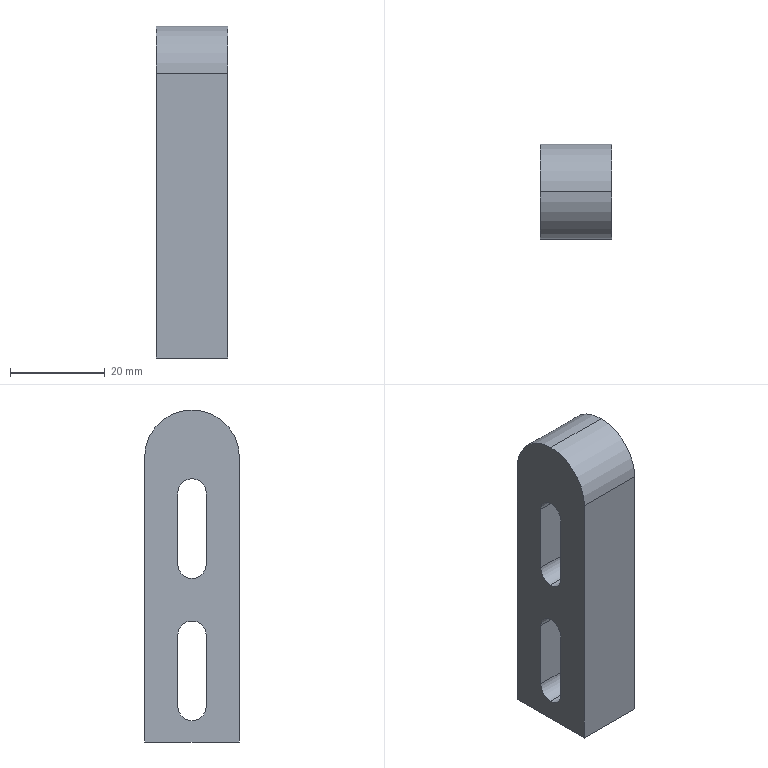Component | SolidWorks | GuideMechanism-1_LimitPlate1-1 | 1 solid | 29 faces | box 15 x 20 x 70 mm | volume 16005 mm3 | plane 15 | cylinder 14 | commonest cylinder face diameters 9 x6 6 x6 20 x2
build123d program:
from build123d import *

# Parameters (mm, degrees)
SKETCH1_W           = 70
SKETCH1_H           = 20
BOSS_EXTRUDE1_DEPTH = 15
FILLET1_RADIUS      = 10
FILLET1_LENGTH      = 15
CUT_EXTRUDE1_DEPTH  = 40.37
CUT_EXTRUDE2_DEPTH  = 5


with BuildPart() as part:
    # Sketch1 → Boss-Extrude1 (new body)
    with BuildSketch(Plane.XY):
        Rectangle(SKETCH1_W, SKETCH1_H)
    extrude(amount=BOSS_EXTRUDE1_DEPTH)

    # Fillet1: full round fillet: the end face becomes a half cylinder, R = half its width
    fillet1_face = Plane((-35, 0, 7.5), x_dir=(0, 0, 1), z_dir=(-1, 0, 0))  # on the end face: x along it, z out of the body
    fillet1_slab = fillet1_face.offset(-FILLET1_RADIUS / 2) * Box(FILLET1_LENGTH, 2 * FILLET1_RADIUS, FILLET1_RADIUS, mode=Mode.PRIVATE)  # the body's end, R deep
    fillet1_round = Plane((-25, 0, 7.5), x_dir=(-1, 0, 0), z_dir=(0, 0, 1)) * Cylinder(FILLET1_RADIUS, FILLET1_LENGTH, mode=Mode.PRIVATE)  # its axis R under the face
    add(fillet1_slab - fillet1_round, mode=Mode.SUBTRACT)

    # Sketch4 → Cut-Extrude1 (cut, through all)
    with BuildSketch(Plane.XY.offset(15)):
        with BuildLine():
            Line((-17.5, 3), (-2.5, 3))
            ThreePointArc((-2.5, 3), (0.5, 0), (-2.5, -3))
            Line((-2.5, -3), (-17.5, -3))
            ThreePointArc((-17.5, -3), (-20.5, 0), (-17.5, 3))
        make_face()
        with BuildLine():
            Line((12.5, 3), (27.5, 3))
            ThreePointArc((27.5, 3), (30.5, 0), (27.5, -3))
            Line((27.5, -3), (12.5, -3))
            ThreePointArc((12.5, -3), (9.5, 0), (12.5, 3))
        make_face()
    extrude(amount=-CUT_EXTRUDE1_DEPTH, mode=Mode.SUBTRACT)

    # Sketch5 → Cut-Extrude2 (cut)
    with BuildSketch(Plane.XY.offset(15)):
        with BuildLine():
            Line((-17.5, 4.5), (-2.5, 4.5))
            ThreePointArc((-2.5, 4.5), (2, 0), (-2.5, -4.5))
            Line((-2.5, -4.5), (-17.5, -4.5))
            ThreePointArc((-17.5, -4.5), (-22, 0), (-17.5, 4.5))
        make_face()
        with BuildLine():
            Line((12.5, 4.5), (27.5, 4.5))
            ThreePointArc((27.5, 4.5), (32, 0), (27.5, -4.5))
            Line((27.5, -4.5), (12.5, -4.5))
            ThreePointArc((12.5, -4.5), (8, 0), (12.5, 4.5))
        make_face()
    extrude(amount=-CUT_EXTRUDE2_DEPTH, mode=Mode.SUBTRACT)


solid = part.part

# Placed as in the assembly
solid = solid.moved(Location((-513.272, -588.766, 1357), (0, 90, 0)))
STEP:
#1=COLOUR_RGB('',0.7922,0.8196,0.9333);
#2=FILL_AREA_STYLE_COLOUR('',#1);
#3=FILL_AREA_STYLE('',(#2));
#4=SURFACE_STYLE_FILL_AREA(#3);
#5=SURFACE_SIDE_STYLE('',(#4));
#6=SURFACE_STYLE_USAGE(.BOTH.,#5);
#7=PRESENTATION_STYLE_ASSIGNMENT((#6));
#8=CARTESIAN_POINT('',(-19.814,-23.18,52.165));
#9=VERTEX_POINT('',#8);
#10=CARTESIAN_POINT('',(-19.814,-23.003,52.343));
#11=VERTEX_POINT('',#10);
#12=CARTESIAN_POINT('',(-19.814,-23.18,52.343));
#13=DIRECTION('',(1.,0.,0.));
#14=DIRECTION('',(0.,0.,-1.));
#15=AXIS2_PLACEMENT_3D('',#12,#13,#14);
#16=CIRCLE('',#15,0.1772);
#17=EDGE_CURVE('',#9,#11,#16,.T.);
#18=ORIENTED_EDGE('',*,*,#17,.F.);
#19=CARTESIAN_POINT('',(-19.617,-23.18,52.165));
#20=VERTEX_POINT('',#19);
#21=CARTESIAN_POINT('',(-19.814,-23.18,52.165));
#22=DIRECTION('',(1.,0.,0.));
#23=VECTOR('',#22,39.37);
#24=LINE('',#21,#23);
#25=EDGE_CURVE('',#9,#20,#24,.T.);
#26=ORIENTED_EDGE('',*,*,#25,.T.);
#27=CARTESIAN_POINT('',(-19.617,-23.003,52.343));
#28=VERTEX_POINT('',#27);
#29=CARTESIAN_POINT('',(-19.617,-23.18,52.343));
#30=DIRECTION('',(1.,0.,0.));
#31=DIRECTION('',(0.,0.,-1.));
#32=AXIS2_PLACEMENT_3D('',#29,#30,#31);
#33=CIRCLE('',#32,0.1772);
#34=EDGE_CURVE('',#20,#28,#33,.T.);
#35=ORIENTED_EDGE('',*,*,#34,.T.);
#36=CARTESIAN_POINT('',(-19.814,-23.003,52.343));
#37=DIRECTION('',(1.,0.,0.));
#38=VECTOR('',#37,39.37);
#39=LINE('',#36,#38);
#40=EDGE_CURVE('',#11,#28,#39,.T.);
#41=ORIENTED_EDGE('',*,*,#40,.F.);
#42=EDGE_LOOP('',(#18,#26,#35,#41));
#43=FACE_OUTER_BOUND('',#42,.T.);
#44=CARTESIAN_POINT('',(-19.814,-23.18,52.343));
#45=DIRECTION('',(1.,0.,0.));
#46=DIRECTION('',(0.,0.,-1.));
#47=AXIS2_PLACEMENT_3D('',#44,#45,#46);
#48=CYLINDRICAL_SURFACE('',#47,0.1772);
#49=ADVANCED_FACE('',(#43),#48,.F.);
#50=CARTESIAN_POINT('',(-19.814,-23.18,53.346));
#51=VERTEX_POINT('',#50);
#52=CARTESIAN_POINT('',(-19.814,-23.003,53.524));
#53=VERTEX_POINT('',#52);
#54=CARTESIAN_POINT('',(-19.814,-23.18,53.524));
#55=DIRECTION('',(1.,0.,0.));
#56=DIRECTION('',(0.,0.,-1.));
#57=AXIS2_PLACEMENT_3D('',#54,#55,#56);
#58=CIRCLE('',#57,0.1772);
#59=EDGE_CURVE('',#51,#53,#58,.T.);
#60=ORIENTED_EDGE('',*,*,#59,.F.);
#61=CARTESIAN_POINT('',(-19.617,-23.18,53.346));
#62=VERTEX_POINT('',#61);
#63=CARTESIAN_POINT('',(-19.814,-23.18,53.346));
#64=DIRECTION('',(1.,0.,0.));
#65=VECTOR('',#64,39.37);
#66=LINE('',#63,#65);
#67=EDGE_CURVE('',#51,#62,#66,.T.);
#68=ORIENTED_EDGE('',*,*,#67,.T.);
#69=CARTESIAN_POINT('',(-19.617,-23.003,53.524));
#70=VERTEX_POINT('',#69);
#71=CARTESIAN_POINT('',(-19.617,-23.18,53.524));
#72=DIRECTION('',(1.,0.,0.));
#73=DIRECTION('',(0.,0.,-1.));
#74=AXIS2_PLACEMENT_3D('',#71,#72,#73);
#75=CIRCLE('',#74,0.1772);
#76=EDGE_CURVE('',#62,#70,#75,.T.);
#77=ORIENTED_EDGE('',*,*,#76,.T.);
#78=CARTESIAN_POINT('',(-19.814,-23.003,53.524));
#79=DIRECTION('',(1.,0.,0.));
#80=VECTOR('',#79,39.37);
#81=LINE('',#78,#80);
#82=EDGE_CURVE('',#53,#70,#81,.T.);
#83=ORIENTED_EDGE('',*,*,#82,.F.);
#84=EDGE_LOOP('',(#60,#68,#77,#83));
#85=FACE_OUTER_BOUND('',#84,.T.);
#86=CARTESIAN_POINT('',(-19.814,-23.18,53.524));
#87=DIRECTION('',(1.,0.,0.));
#88=DIRECTION('',(0.,0.,-1.));
#89=AXIS2_PLACEMENT_3D('',#86,#87,#88);
#90=CYLINDRICAL_SURFACE('',#89,0.1772);
#91=ADVANCED_FACE('',(#85),#90,.F.);
#92=CARTESIAN_POINT('',(-19.617,-23.18,54.803));
#93=VERTEX_POINT('',#92);
#94=CARTESIAN_POINT('',(-19.617,-23.573,54.409));
#95=VERTEX_POINT('',#94);
#96=CARTESIAN_POINT('',(-19.617,-23.18,54.409));
#97=DIRECTION('',(1.,0.,0.));
#98=DIRECTION('',(0.,0.,1.));
#99=AXIS2_PLACEMENT_3D('',#96,#97,#98);
#100=CIRCLE('',#99,0.3937);
#101=EDGE_CURVE('',#93,#95,#100,.T.);
#102=ORIENTED_EDGE('',*,*,#101,.F.);
#103=CARTESIAN_POINT('',(-20.208,-23.18,54.803));
#104=VERTEX_POINT('',#103);
#105=CARTESIAN_POINT('',(-20.208,-23.18,54.803));
#106=DIRECTION('',(-1.,0.,0.));
#107=VECTOR('',#106,39.37);
#108=LINE('',#105,#107);
#109=EDGE_CURVE('',#93,#104,#108,.T.);
#110=ORIENTED_EDGE('',*,*,#109,.T.);
#111=CARTESIAN_POINT('',(-20.208,-23.573,54.409));
#112=VERTEX_POINT('',#111);
#113=CARTESIAN_POINT('',(-20.208,-23.18,54.409));
#114=DIRECTION('',(-1.,0.,0.));
#115=DIRECTION('',(0.,0.,1.));
#116=AXIS2_PLACEMENT_3D('',#113,#114,#115);
#117=CIRCLE('',#116,0.3937);
#118=EDGE_CURVE('',#112,#104,#117,.T.);
#119=ORIENTED_EDGE('',*,*,#118,.F.);
#120=CARTESIAN_POINT('',(-19.617,-23.573,54.409));
#121=DIRECTION('',(-1.,0.,0.));
#122=VECTOR('',#121,39.37);
#123=LINE('',#120,#122);
#124=EDGE_CURVE('',#95,#112,#123,.T.);
#125=ORIENTED_EDGE('',*,*,#124,.F.);
#126=EDGE_LOOP('',(#102,#110,#119,#125));
#127=FACE_OUTER_BOUND('',#126,.T.);
#128=CARTESIAN_POINT('',(-20.208,-23.18,54.409));
#129=DIRECTION('',(-1.,0.,0.));
#130=DIRECTION('',(0.,0.,1.));
#131=AXIS2_PLACEMENT_3D('',#128,#129,#130);
#132=CYLINDRICAL_SURFACE('',#131,0.3937);
#133=ADVANCED_FACE('',(#127),#132,.T.);
#134=CARTESIAN_POINT('',(-20.208,-23.18,53.406));
#135=VERTEX_POINT('',#134);
#136=CARTESIAN_POINT('',(-20.208,-23.062,53.524));
#137=VERTEX_POINT('',#136);
#138=CARTESIAN_POINT('',(-20.208,-23.18,53.524));
#139=DIRECTION('',(1.,0.,0.));
#140=DIRECTION('',(0.,0.,-1.));
#141=AXIS2_PLACEMENT_3D('',#138,#139,#140);
#142=CIRCLE('',#141,0.1181);
#143=EDGE_CURVE('',#135,#137,#142,.T.);
#144=ORIENTED_EDGE('',*,*,#143,.F.);
#145=CARTESIAN_POINT('',(-19.814,-23.18,53.406));
#146=VERTEX_POINT('',#145);
#147=CARTESIAN_POINT('',(-20.208,-23.18,53.406));
#148=DIRECTION('',(1.,0.,0.));
#149=VECTOR('',#148,39.37);
#150=LINE('',#147,#149);
#151=EDGE_CURVE('',#135,#146,#150,.T.);
#152=ORIENTED_EDGE('',*,*,#151,.T.);
#153=CARTESIAN_POINT('',(-19.814,-23.062,53.524));
#154=VERTEX_POINT('',#153);
#155=CARTESIAN_POINT('',(-19.814,-23.18,53.524));
#156=DIRECTION('',(-1.,0.,0.));
#157=DIRECTION('',(0.,0.,-1.));
#158=AXIS2_PLACEMENT_3D('',#155,#156,#157);
#159=CIRCLE('',#158,0.1181);
#160=EDGE_CURVE('',#154,#146,#159,.T.);
#161=ORIENTED_EDGE('',*,*,#160,.F.);
#162=CARTESIAN_POINT('',(-20.208,-23.062,53.524));
#163=DIRECTION('',(1.,0.,0.));
#164=VECTOR('',#163,39.37);
#165=LINE('',#162,#164);
#166=EDGE_CURVE('',#137,#154,#165,.T.);
#167=ORIENTED_EDGE('',*,*,#166,.F.);
#168=EDGE_LOOP('',(#144,#152,#161,#167));
#169=FACE_OUTER_BOUND('',#168,.T.);
#170=CARTESIAN_POINT('',(-20.208,-23.18,53.524));
#171=DIRECTION('',(1.,0.,0.));
#172=DIRECTION('',(0.,0.,-1.));
#173=AXIS2_PLACEMENT_3D('',#170,#171,#172);
#174=CYLINDRICAL_SURFACE('',#173,0.1181);
#175=ADVANCED_FACE('',(#169),#174,.F.);
#176=CARTESIAN_POINT('',(-20.208,-23.18,52.224));
#177=VERTEX_POINT('',#176);
#178=CARTESIAN_POINT('',(-20.208,-23.062,52.343));
#179=VERTEX_POINT('',#178);
#180=CARTESIAN_POINT('',(-20.208,-23.18,52.343));
#181=DIRECTION('',(1.,0.,0.));
#182=DIRECTION('',(0.,0.,-1.));
#183=AXIS2_PLACEMENT_3D('',#180,#181,#182);
#184=CIRCLE('',#183,0.1181);
#185=EDGE_CURVE('',#177,#179,#184,.T.);
#186=ORIENTED_EDGE('',*,*,#185,.F.);
#187=CARTESIAN_POINT('',(-19.814,-23.18,52.224));
#188=VERTEX_POINT('',#187);
#189=CARTESIAN_POINT('',(-20.208,-23.18,52.224));
#190=DIRECTION('',(1.,0.,0.));
#191=VECTOR('',#190,39.37);
#192=LINE('',#189,#191);
#193=EDGE_CURVE('',#177,#188,#192,.T.);
#194=ORIENTED_EDGE('',*,*,#193,.T.);
#195=CARTESIAN_POINT('',(-19.814,-23.062,52.343));
#196=VERTEX_POINT('',#195);
#197=CARTESIAN_POINT('',(-19.814,-23.18,52.343));
#198=DIRECTION('',(-1.,0.,0.));
#199=DIRECTION('',(0.,0.,-1.));
#200=AXIS2_PLACEMENT_3D('',#197,#198,#199);
#201=CIRCLE('',#200,0.1181);
#202=EDGE_CURVE('',#196,#188,#201,.T.);
#203=ORIENTED_EDGE('',*,*,#202,.F.);
#204=CARTESIAN_POINT('',(-20.208,-23.062,52.343));
#205=DIRECTION('',(1.,0.,0.));
#206=VECTOR('',#205,39.37);
#207=LINE('',#204,#206);
#208=EDGE_CURVE('',#179,#196,#207,.T.);
#209=ORIENTED_EDGE('',*,*,#208,.F.);
#210=EDGE_LOOP('',(#186,#194,#203,#209));
#211=FACE_OUTER_BOUND('',#210,.T.);
#212=CARTESIAN_POINT('',(-20.208,-23.18,52.343));
#213=DIRECTION('',(1.,0.,0.));
#214=DIRECTION('',(0.,0.,-1.));
#215=AXIS2_PLACEMENT_3D('',#212,#213,#214);
#216=CYLINDRICAL_SURFACE('',#215,0.1181);
#217=ADVANCED_FACE('',(#211),#216,.F.);
#218=CARTESIAN_POINT('',(-19.814,-23.298,52.933));
#219=VERTEX_POINT('',#218);
#220=CARTESIAN_POINT('',(-19.814,-23.062,52.933));
#221=VERTEX_POINT('',#220);
#222=CARTESIAN_POINT('',(-19.814,-23.18,52.933));
#223=DIRECTION('',(-1.,0.,0.));
#224=DIRECTION('',(0.,0.,-1.));
#225=AXIS2_PLACEMENT_3D('',#222,#223,#224);
#226=CIRCLE('',#225,0.1181);
#227=EDGE_CURVE('',#219,#221,#226,.T.);
#228=ORIENTED_EDGE('',*,*,#227,.F.);
#229=CARTESIAN_POINT('',(-20.208,-23.298,52.933));
#230=VERTEX_POINT('',#229);
#231=CARTESIAN_POINT('',(-20.208,-23.298,52.933));
#232=DIRECTION('',(1.,0.,0.));
#233=VECTOR('',#232,39.37);
#234=LINE('',#231,#233);
#235=EDGE_CURVE('',#230,#219,#234,.T.);
#236=ORIENTED_EDGE('',*,*,#235,.F.);
#237=CARTESIAN_POINT('',(-20.208,-23.062,52.933));
#238=VERTEX_POINT('',#237);
#239=CARTESIAN_POINT('',(-20.208,-23.18,52.933));
#240=DIRECTION('',(1.,0.,0.));
#241=DIRECTION('',(0.,0.,-1.));
#242=AXIS2_PLACEMENT_3D('',#239,#240,#241);
#243=CIRCLE('',#242,0.1181);
#244=EDGE_CURVE('',#238,#230,#243,.T.);
#245=ORIENTED_EDGE('',*,*,#244,.F.);
#246=CARTESIAN_POINT('',(-20.208,-23.062,52.933));
#247=DIRECTION('',(1.,0.,0.));
#248=VECTOR('',#247,39.37);
#249=LINE('',#246,#248);
#250=EDGE_CURVE('',#238,#221,#249,.T.);
#251=ORIENTED_EDGE('',*,*,#250,.T.);
#252=EDGE_LOOP('',(#228,#236,#245,#251));
#253=FACE_OUTER_BOUND('',#252,.T.);
#254=CARTESIAN_POINT('',(-20.208,-23.18,52.933));
#255=DIRECTION('',(1.,0.,0.));
#256=DIRECTION('',(0.,0.,-1.));
#257=AXIS2_PLACEMENT_3D('',#254,#255,#256);
#258=CYLINDRICAL_SURFACE('',#257,0.1181);
#259=ADVANCED_FACE('',(#253),#258,.F.);
#260=CARTESIAN_POINT('',(-19.814,-23.062,52.933));
#261=DIRECTION('',(0.,0.,-1.));
#262=VECTOR('',#261,39.37);
#263=LINE('',#260,#262);
#264=EDGE_CURVE('',#221,#196,#263,.T.);
#265=ORIENTED_EDGE('',*,*,#264,.F.);
#266=ORIENTED_EDGE('',*,*,#250,.F.);
#267=CARTESIAN_POINT('',(-20.208,-23.062,52.933));
#268=DIRECTION('',(0.,-0.,1.));
#269=VECTOR('',#268,39.37);
#270=LINE('',#267,#269);
#271=EDGE_CURVE('',#179,#238,#270,.T.);
#272=ORIENTED_EDGE('',*,*,#271,.F.);
#273=ORIENTED_EDGE('',*,*,#208,.T.);
#274=EDGE_LOOP('',(#265,#266,#272,#273));
#275=FACE_OUTER_BOUND('',#274,.T.);
#276=CARTESIAN_POINT('',(-20.208,-23.062,52.933));
#277=DIRECTION('',(0.,1.,0.));
#278=DIRECTION('',(0.,-0.,1.));
#279=AXIS2_PLACEMENT_3D('',#276,#277,#278);
#280=PLANE('',#279);
#281=ADVANCED_FACE('',(#275),#280,.F.);
#282=ORIENTED_EDGE('',*,*,#193,.F.);
#283=CARTESIAN_POINT('',(-20.208,-23.298,52.343));
#284=VERTEX_POINT('',#283);
#285=CARTESIAN_POINT('',(-20.208,-23.18,52.343));
#286=DIRECTION('',(1.,0.,0.));
#287=DIRECTION('',(0.,0.,-1.));
#288=AXIS2_PLACEMENT_3D('',#285,#286,#287);
#289=CIRCLE('',#288,0.1181);
#290=EDGE_CURVE('',#284,#177,#289,.T.);
#291=ORIENTED_EDGE('',*,*,#290,.F.);
#292=CARTESIAN_POINT('',(-19.814,-23.298,52.343));
#293=VERTEX_POINT('',#292);
#294=CARTESIAN_POINT('',(-20.208,-23.298,52.343));
#295=DIRECTION('',(1.,0.,0.));
#296=VECTOR('',#295,39.37);
#297=LINE('',#294,#296);
#298=EDGE_CURVE('',#284,#293,#297,.T.);
#299=ORIENTED_EDGE('',*,*,#298,.T.);
#300=CARTESIAN_POINT('',(-19.814,-23.18,52.343));
#301=DIRECTION('',(-1.,0.,0.));
#302=DIRECTION('',(0.,0.,-1.));
#303=AXIS2_PLACEMENT_3D('',#300,#301,#302);
#304=CIRCLE('',#303,0.1181);
#305=EDGE_CURVE('',#188,#293,#304,.T.);
#306=ORIENTED_EDGE('',*,*,#305,.F.);
#307=EDGE_LOOP('',(#282,#291,#299,#306));
#308=FACE_OUTER_BOUND('',#307,.T.);
#309=CARTESIAN_POINT('',(-20.208,-23.18,52.343));
#310=DIRECTION('',(1.,0.,0.));
#311=DIRECTION('',(0.,0.,-1.));
#312=AXIS2_PLACEMENT_3D('',#309,#310,#311);
#313=CYLINDRICAL_SURFACE('',#312,0.1181);
#314=ADVANCED_FACE('',(#308),#313,.F.);
#315=CARTESIAN_POINT('',(-19.814,-23.298,52.933));
#316=DIRECTION('',(0.,-0.,1.));
#317=VECTOR('',#316,39.37);
#318=LINE('',#315,#317);
#319=EDGE_CURVE('',#293,#219,#318,.T.);
#320=ORIENTED_EDGE('',*,*,#319,.F.);
#321=ORIENTED_EDGE('',*,*,#298,.F.);
#322=CARTESIAN_POINT('',(-20.208,-23.298,52.933));
#323=DIRECTION('',(0.,0.,-1.));
#324=VECTOR('',#323,39.37);
#325=LINE('',#322,#324);
#326=EDGE_CURVE('',#230,#284,#325,.T.);
#327=ORIENTED_EDGE('',*,*,#326,.F.);
#328=ORIENTED_EDGE('',*,*,#235,.T.);
#329=EDGE_LOOP('',(#320,#321,#327,#328));
#330=FACE_OUTER_BOUND('',#329,.T.);
#331=CARTESIAN_POINT('',(-20.208,-23.298,52.933));
#332=DIRECTION('',(0.,-1.,-0.));
#333=DIRECTION('',(0.,0.,-1.));
#334=AXIS2_PLACEMENT_3D('',#331,#332,#333);
#335=PLANE('',#334);
#336=ADVANCED_FACE('',(#330),#335,.F.);
#337=CARTESIAN_POINT('',(-19.814,-23.298,54.114));
#338=VERTEX_POINT('',#337);
#339=CARTESIAN_POINT('',(-19.814,-23.062,54.114));
#340=VERTEX_POINT('',#339);
#341=CARTESIAN_POINT('',(-19.814,-23.18,54.114));
#342=DIRECTION('',(-1.,0.,0.));
#343=DIRECTION('',(0.,0.,-1.));
#344=AXIS2_PLACEMENT_3D('',#341,#342,#343);
#345=CIRCLE('',#344,0.1181);
#346=EDGE_CURVE('',#338,#340,#345,.T.);
#347=ORIENTED_EDGE('',*,*,#346,.F.);
#348=CARTESIAN_POINT('',(-20.208,-23.298,54.114));
#349=VERTEX_POINT('',#348);
#350=CARTESIAN_POINT('',(-20.208,-23.298,54.114));
#351=DIRECTION('',(1.,0.,0.));
#352=VECTOR('',#351,39.37);
#353=LINE('',#350,#352);
#354=EDGE_CURVE('',#349,#338,#353,.T.);
#355=ORIENTED_EDGE('',*,*,#354,.F.);
#356=CARTESIAN_POINT('',(-20.208,-23.062,54.114));
#357=VERTEX_POINT('',#356);
#358=CARTESIAN_POINT('',(-20.208,-23.18,54.114));
#359=DIRECTION('',(1.,0.,0.));
#360=DIRECTION('',(0.,0.,-1.));
#361=AXIS2_PLACEMENT_3D('',#358,#359,#360);
#362=CIRCLE('',#361,0.1181);
#363=EDGE_CURVE('',#357,#349,#362,.T.);
#364=ORIENTED_EDGE('',*,*,#363,.F.);
#365=CARTESIAN_POINT('',(-20.208,-23.062,54.114));
#366=DIRECTION('',(1.,0.,0.));
#367=VECTOR('',#366,39.37);
#368=LINE('',#365,#367);
#369=EDGE_CURVE('',#357,#340,#368,.T.);
#370=ORIENTED_EDGE('',*,*,#369,.T.);
#371=EDGE_LOOP('',(#347,#355,#364,#370));
#372=FACE_OUTER_BOUND('',#371,.T.);
#373=CARTESIAN_POINT('',(-20.208,-23.18,54.114));
#374=DIRECTION('',(1.,0.,0.));
#375=DIRECTION('',(0.,0.,-1.));
#376=AXIS2_PLACEMENT_3D('',#373,#374,#375);
#377=CYLINDRICAL_SURFACE('',#376,0.1181);
#378=ADVANCED_FACE('',(#372),#377,.F.);
#379=CARTESIAN_POINT('',(-19.814,-23.062,54.114));
#380=DIRECTION('',(0.,0.,-1.));
#381=VECTOR('',#380,39.37);
#382=LINE('',#379,#381);
#383=EDGE_CURVE('',#340,#154,#382,.T.);
#384=ORIENTED_EDGE('',*,*,#383,.F.);
#385=ORIENTED_EDGE('',*,*,#369,.F.);
#386=CARTESIAN_POINT('',(-20.208,-23.062,54.114));
#387=DIRECTION('',(0.,-0.,1.));
#388=VECTOR('',#387,39.37);
#389=LINE('',#386,#388);
#390=EDGE_CURVE('',#137,#357,#389,.T.);
#391=ORIENTED_EDGE('',*,*,#390,.F.);
#392=ORIENTED_EDGE('',*,*,#166,.T.);
#393=EDGE_LOOP('',(#384,#385,#391,#392));
#394=FACE_OUTER_BOUND('',#393,.T.);
#395=CARTESIAN_POINT('',(-20.208,-23.062,54.114));
#396=DIRECTION('',(0.,1.,0.));
#397=DIRECTION('',(0.,-0.,1.));
#398=AXIS2_PLACEMENT_3D('',#395,#396,#397);
#399=PLANE('',#398);
#400=ADVANCED_FACE('',(#394),#399,.F.);
#401=ORIENTED_EDGE('',*,*,#151,.F.);
#402=CARTESIAN_POINT('',(-20.208,-23.298,53.524));
#403=VERTEX_POINT('',#402);
#404=CARTESIAN_POINT('',(-20.208,-23.18,53.524));
#405=DIRECTION('',(1.,0.,0.));
#406=DIRECTION('',(0.,0.,-1.));
#407=AXIS2_PLACEMENT_3D('',#404,#405,#406);
#408=CIRCLE('',#407,0.1181);
#409=EDGE_CURVE('',#403,#135,#408,.T.);
#410=ORIENTED_EDGE('',*,*,#409,.F.);
#411=CARTESIAN_POINT('',(-19.814,-23.298,53.524));
#412=VERTEX_POINT('',#411);
#413=CARTESIAN_POINT('',(-20.208,-23.298,53.524));
#414=DIRECTION('',(1.,0.,0.));
#415=VECTOR('',#414,39.37);
#416=LINE('',#413,#415);
#417=EDGE_CURVE('',#403,#412,#416,.T.);
#418=ORIENTED_EDGE('',*,*,#417,.T.);
#419=CARTESIAN_POINT('',(-19.814,-23.18,53.524));
#420=DIRECTION('',(-1.,0.,0.));
#421=DIRECTION('',(0.,0.,-1.));
#422=AXIS2_PLACEMENT_3D('',#419,#420,#421);
#423=CIRCLE('',#422,0.1181);
#424=EDGE_CURVE('',#146,#412,#423,.T.);
#425=ORIENTED_EDGE('',*,*,#424,.F.);
#426=EDGE_LOOP('',(#401,#410,#418,#425));
#427=FACE_OUTER_BOUND('',#426,.T.);
#428=CARTESIAN_POINT('',(-20.208,-23.18,53.524));
#429=DIRECTION('',(1.,0.,0.));
#430=DIRECTION('',(0.,0.,-1.));
#431=AXIS2_PLACEMENT_3D('',#428,#429,#430);
#432=CYLINDRICAL_SURFACE('',#431,0.1181);
#433=ADVANCED_FACE('',(#427),#432,.F.);
#434=CARTESIAN_POINT('',(-19.814,-23.298,54.114));
#435=DIRECTION('',(0.,-0.,1.));
#436=VECTOR('',#435,39.37);
#437=LINE('',#434,#436);
#438=EDGE_CURVE('',#412,#338,#437,.T.);
#439=ORIENTED_EDGE('',*,*,#438,.F.);
#440=ORIENTED_EDGE('',*,*,#417,.F.);
#441=CARTESIAN_POINT('',(-20.208,-23.298,54.114));
#442=DIRECTION('',(0.,0.,-1.));
#443=VECTOR('',#442,39.37);
#444=LINE('',#441,#443);
#445=EDGE_CURVE('',#349,#403,#444,.T.);
#446=ORIENTED_EDGE('',*,*,#445,.F.);
#447=ORIENTED_EDGE('',*,*,#354,.T.);
#448=EDGE_LOOP('',(#439,#440,#446,#447));
#449=FACE_OUTER_BOUND('',#448,.T.);
#450=CARTESIAN_POINT('',(-20.208,-23.298,54.114));
#451=DIRECTION('',(0.,-1.,-0.));
#452=DIRECTION('',(0.,0.,-1.));
#453=AXIS2_PLACEMENT_3D('',#450,#451,#452);
#454=PLANE('',#453);
#455=ADVANCED_FACE('',(#449),#454,.F.);
#456=ORIENTED_EDGE('',*,*,#109,.F.);
#457=CARTESIAN_POINT('',(-19.617,-22.786,54.409));
#458=VERTEX_POINT('',#457);
#459=CARTESIAN_POINT('',(-19.617,-23.18,54.409));
#460=DIRECTION('',(1.,0.,0.));
#461=DIRECTION('',(0.,0.,1.));
#462=AXIS2_PLACEMENT_3D('',#459,#460,#461);
#463=CIRCLE('',#462,0.3937);
#464=EDGE_CURVE('',#458,#93,#463,.T.);
#465=ORIENTED_EDGE('',*,*,#464,.F.);
#466=CARTESIAN_POINT('',(-20.208,-22.786,54.409));
#467=VERTEX_POINT('',#466);
#468=CARTESIAN_POINT('',(-19.617,-22.786,54.409));
#469=DIRECTION('',(1.,0.,0.));
#470=VECTOR('',#469,39.37);
#471=LINE('',#468,#470);
#472=EDGE_CURVE('',#467,#458,#471,.T.);
#473=ORIENTED_EDGE('',*,*,#472,.F.);
#474=CARTESIAN_POINT('',(-20.208,-23.18,54.409));
#475=DIRECTION('',(-1.,0.,0.));
#476=DIRECTION('',(0.,0.,1.));
#477=AXIS2_PLACEMENT_3D('',#474,#475,#476);
#478=CIRCLE('',#477,0.3937);
#479=EDGE_CURVE('',#104,#467,#478,.T.);
#480=ORIENTED_EDGE('',*,*,#479,.F.);
#481=EDGE_LOOP('',(#456,#465,#473,#480));
#482=FACE_OUTER_BOUND('',#481,.T.);
#483=CARTESIAN_POINT('',(-20.208,-23.18,54.409));
#484=DIRECTION('',(-1.,0.,0.));
#485=DIRECTION('',(0.,0.,1.));
#486=AXIS2_PLACEMENT_3D('',#483,#484,#485);
#487=CYLINDRICAL_SURFACE('',#486,0.3937);
#488=ADVANCED_FACE('',(#482),#487,.T.);
#489=CARTESIAN_POINT('',(-20.208,-23.573,52.047));
#490=VERTEX_POINT('',#489);
#491=CARTESIAN_POINT('',(-20.208,-22.786,52.047));
#492=VERTEX_POINT('',#491);
#493=CARTESIAN_POINT('',(-20.208,-23.573,52.047));
#494=DIRECTION('',(0.,1.,0.));
#495=VECTOR('',#494,39.37);
#496=LINE('',#493,#495);
#497=EDGE_CURVE('',#490,#492,#496,.T.);
#498=ORIENTED_EDGE('',*,*,#497,.T.);
#499=CARTESIAN_POINT('',(-19.617,-22.786,52.047));
#500=VERTEX_POINT('',#499);
#501=CARTESIAN_POINT('',(-19.617,-22.786,52.047));
#502=DIRECTION('',(-1.,0.,0.));
#503=VECTOR('',#502,39.37);
#504=LINE('',#501,#503);
#505=EDGE_CURVE('',#500,#492,#504,.T.);
#506=ORIENTED_EDGE('',*,*,#505,.F.);
#507=CARTESIAN_POINT('',(-19.617,-23.573,52.047));
#508=VERTEX_POINT('',#507);
#509=CARTESIAN_POINT('',(-19.617,-23.573,52.047));
#510=DIRECTION('',(0.,1.,0.));
#511=VECTOR('',#510,39.37);
#512=LINE('',#509,#511);
#513=EDGE_CURVE('',#508,#500,#512,.T.);
#514=ORIENTED_EDGE('',*,*,#513,.F.);
#515=CARTESIAN_POINT('',(-19.617,-23.573,52.047));
#516=DIRECTION('',(-1.,0.,0.));
#517=VECTOR('',#516,39.37);
#518=LINE('',#515,#517);
#519=EDGE_CURVE('',#508,#490,#518,.T.);
#520=ORIENTED_EDGE('',*,*,#519,.T.);
#521=EDGE_LOOP('',(#498,#506,#514,#520));
#522=FACE_OUTER_BOUND('',#521,.T.);
#523=CARTESIAN_POINT('',(-19.617,-23.573,52.047));
#524=DIRECTION('',(0.,0.,1.));
#525=DIRECTION('',(1.,0.,0.));
#526=AXIS2_PLACEMENT_3D('',#523,#524,#525);
#527=PLANE('',#526);
#528=ADVANCED_FACE('',(#522),#527,.F.);
#529=CARTESIAN_POINT('',(-20.208,-22.786,54.803));
#530=DIRECTION('',(0.,0.,1.));
#531=VECTOR('',#530,39.37);
#532=LINE('',#529,#531);
#533=EDGE_CURVE('',#492,#467,#532,.T.);
#534=ORIENTED_EDGE('',*,*,#533,.T.);
#535=ORIENTED_EDGE('',*,*,#472,.T.);
#536=CARTESIAN_POINT('',(-19.617,-22.786,54.803));
#537=DIRECTION('',(0.,0.,1.));
#538=VECTOR('',#537,39.37);
#539=LINE('',#536,#538);
#540=EDGE_CURVE('',#500,#458,#539,.T.);
#541=ORIENTED_EDGE('',*,*,#540,.F.);
#542=ORIENTED_EDGE('',*,*,#505,.T.);
#543=EDGE_LOOP('',(#534,#535,#541,#542));
#544=FACE_OUTER_BOUND('',#543,.T.);
#545=CARTESIAN_POINT('',(-19.617,-22.786,54.803));
#546=DIRECTION('',(0.,-1.,0.));
#547=DIRECTION('',(-1.,0.,0.));
#548=AXIS2_PLACEMENT_3D('',#545,#546,#547);
#549=PLANE('',#548);
#550=ADVANCED_FACE('',(#544),#549,.F.);
#551=CARTESIAN_POINT('',(-19.617,-23.573,54.803));
#552=DIRECTION('',(0.,0.,-1.));
#553=VECTOR('',#552,39.37);
#554=LINE('',#551,#553);
#555=EDGE_CURVE('',#95,#508,#554,.T.);
#556=ORIENTED_EDGE('',*,*,#555,.F.);
#557=ORIENTED_EDGE('',*,*,#124,.T.);
#558=CARTESIAN_POINT('',(-20.208,-23.573,54.803));
#559=DIRECTION('',(0.,0.,-1.));
#560=VECTOR('',#559,39.37);
#561=LINE('',#558,#560);
#562=EDGE_CURVE('',#112,#490,#561,.T.);
#563=ORIENTED_EDGE('',*,*,#562,.T.);
#564=ORIENTED_EDGE('',*,*,#519,.F.);
#565=EDGE_LOOP('',(#556,#557,#563,#564));
#566=FACE_OUTER_BOUND('',#565,.T.);
#567=CARTESIAN_POINT('',(-19.617,-23.573,54.803));
#568=DIRECTION('',(0.,1.,0.));
#569=DIRECTION('',(1.,0.,0.));
#570=AXIS2_PLACEMENT_3D('',#567,#568,#569);
#571=PLANE('',#570);
#572=ADVANCED_FACE('',(#566),#571,.F.);
#573=CARTESIAN_POINT('',(-19.617,-23.357,52.933));
#574=VERTEX_POINT('',#573);
#575=CARTESIAN_POINT('',(-19.617,-23.357,52.343));
#576=VERTEX_POINT('',#575);
#577=CARTESIAN_POINT('',(-19.617,-23.357,52.933));
#578=DIRECTION('',(0.,-0.,-1.));
#579=VECTOR('',#578,39.37);
#580=LINE('',#577,#579);
#581=EDGE_CURVE('',#574,#576,#580,.T.);
#582=ORIENTED_EDGE('',*,*,#581,.F.);
#583=CARTESIAN_POINT('',(-19.617,-23.003,52.933));
#584=VERTEX_POINT('',#583);
#585=CARTESIAN_POINT('',(-19.617,-23.18,52.933));
#586=DIRECTION('',(1.,0.,0.));
#587=DIRECTION('',(0.,0.,-1.));
#588=AXIS2_PLACEMENT_3D('',#585,#586,#587);
#589=CIRCLE('',#588,0.1772);
#590=EDGE_CURVE('',#584,#574,#589,.T.);
#591=ORIENTED_EDGE('',*,*,#590,.F.);
#592=CARTESIAN_POINT('',(-19.617,-23.003,52.933));
#593=DIRECTION('',(0.,-0.,1.));
#594=VECTOR('',#593,39.37);
#595=LINE('',#592,#594);
#596=EDGE_CURVE('',#28,#584,#595,.T.);
#597=ORIENTED_EDGE('',*,*,#596,.F.);
#598=ORIENTED_EDGE('',*,*,#34,.F.);
#599=CARTESIAN_POINT('',(-19.617,-23.18,52.343));
#600=DIRECTION('',(1.,0.,0.));
#601=DIRECTION('',(0.,0.,-1.));
#602=AXIS2_PLACEMENT_3D('',#599,#600,#601);
#603=CIRCLE('',#602,0.1772);
#604=EDGE_CURVE('',#576,#20,#603,.T.);
#605=ORIENTED_EDGE('',*,*,#604,.F.);
#606=EDGE_LOOP('',(#582,#591,#597,#598,#605));
#607=FACE_BOUND('',#606,.T.);
#608=CARTESIAN_POINT('',(-19.617,-23.357,54.114));
#609=VERTEX_POINT('',#608);
#610=CARTESIAN_POINT('',(-19.617,-23.357,53.524));
#611=VERTEX_POINT('',#610);
#612=CARTESIAN_POINT('',(-19.617,-23.357,54.114));
#613=DIRECTION('',(0.,0.,-1.));
#614=VECTOR('',#613,39.37);
#615=LINE('',#612,#614);
#616=EDGE_CURVE('',#609,#611,#615,.T.);
#617=ORIENTED_EDGE('',*,*,#616,.F.);
#618=CARTESIAN_POINT('',(-19.617,-23.003,54.114));
#619=VERTEX_POINT('',#618);
#620=CARTESIAN_POINT('',(-19.617,-23.18,54.114));
#621=DIRECTION('',(1.,0.,0.));
#622=DIRECTION('',(0.,0.,-1.));
#623=AXIS2_PLACEMENT_3D('',#620,#621,#622);
#624=CIRCLE('',#623,0.1772);
#625=EDGE_CURVE('',#619,#609,#624,.T.);
#626=ORIENTED_EDGE('',*,*,#625,.F.);
#627=CARTESIAN_POINT('',(-19.617,-23.003,54.114));
#628=DIRECTION('',(0.,0.,1.));
#629=VECTOR('',#628,39.37);
#630=LINE('',#627,#629);
#631=EDGE_CURVE('',#70,#619,#630,.T.);
#632=ORIENTED_EDGE('',*,*,#631,.F.);
#633=ORIENTED_EDGE('',*,*,#76,.F.);
#634=CARTESIAN_POINT('',(-19.617,-23.18,53.524));
#635=DIRECTION('',(1.,0.,0.));
#636=DIRECTION('',(0.,0.,-1.));
#637=AXIS2_PLACEMENT_3D('',#634,#635,#636);
#638=CIRCLE('',#637,0.1772);
#639=EDGE_CURVE('',#611,#62,#638,.T.);
#640=ORIENTED_EDGE('',*,*,#639,.F.);
#641=EDGE_LOOP('',(#617,#626,#632,#633,#640));
#642=FACE_BOUND('',#641,.T.);
#643=ORIENTED_EDGE('',*,*,#540,.T.);
#644=ORIENTED_EDGE('',*,*,#464,.T.);
#645=ORIENTED_EDGE('',*,*,#101,.T.);
#646=ORIENTED_EDGE('',*,*,#555,.T.);
#647=ORIENTED_EDGE('',*,*,#513,.T.);
#648=EDGE_LOOP('',(#643,#644,#645,#646,#647));
#649=FACE_OUTER_BOUND('',#648,.T.);
#650=CARTESIAN_POINT('',(-19.617,-23.18,53.425));
#651=DIRECTION('',(-1.,0.,0.));
#652=DIRECTION('',(0.,0.,1.));
#653=AXIS2_PLACEMENT_3D('',#650,#651,#652);
#654=PLANE('',#653);
#655=ADVANCED_FACE('',(#607,#642,#649),#654,.F.);
#656=ORIENTED_EDGE('',*,*,#244,.T.);
#657=ORIENTED_EDGE('',*,*,#326,.T.);
#658=ORIENTED_EDGE('',*,*,#290,.T.);
#659=ORIENTED_EDGE('',*,*,#185,.T.);
#660=ORIENTED_EDGE('',*,*,#271,.T.);
#661=EDGE_LOOP('',(#656,#657,#658,#659,#660));
#662=FACE_BOUND('',#661,.T.);
#663=ORIENTED_EDGE('',*,*,#363,.T.);
#664=ORIENTED_EDGE('',*,*,#445,.T.);
#665=ORIENTED_EDGE('',*,*,#409,.T.);
#666=ORIENTED_EDGE('',*,*,#143,.T.);
#667=ORIENTED_EDGE('',*,*,#390,.T.);
#668=EDGE_LOOP('',(#663,#664,#665,#666,#667));
#669=FACE_BOUND('',#668,.T.);
#670=ORIENTED_EDGE('',*,*,#562,.F.);
#671=ORIENTED_EDGE('',*,*,#118,.T.);
#672=ORIENTED_EDGE('',*,*,#479,.T.);
#673=ORIENTED_EDGE('',*,*,#533,.F.);
#674=ORIENTED_EDGE('',*,*,#497,.F.);
#675=EDGE_LOOP('',(#670,#671,#672,#673,#674));
#676=FACE_OUTER_BOUND('',#675,.T.);
#677=CARTESIAN_POINT('',(-20.208,-23.18,53.425));
#678=DIRECTION('',(-1.,0.,0.));
#679=DIRECTION('',(0.,0.,1.));
#680=AXIS2_PLACEMENT_3D('',#677,#678,#679);
#681=PLANE('',#680);
#682=ADVANCED_FACE('',(#662,#669,#676),#681,.T.);
#683=CARTESIAN_POINT('',(-19.814,-23.003,54.114));
#684=VERTEX_POINT('',#683);
#685=CARTESIAN_POINT('',(-19.814,-23.357,54.114));
#686=VERTEX_POINT('',#685);
#687=CARTESIAN_POINT('',(-19.814,-23.18,54.114));
#688=DIRECTION('',(1.,0.,0.));
#689=DIRECTION('',(0.,0.,-1.));
#690=AXIS2_PLACEMENT_3D('',#687,#688,#689);
#691=CIRCLE('',#690,0.1772);
#692=EDGE_CURVE('',#684,#686,#691,.T.);
#693=ORIENTED_EDGE('',*,*,#692,.T.);
#694=CARTESIAN_POINT('',(-19.814,-23.357,53.524));
#695=VERTEX_POINT('',#694);
#696=CARTESIAN_POINT('',(-19.814,-23.357,54.114));
#697=DIRECTION('',(0.,0.,-1.));
#698=VECTOR('',#697,39.37);
#699=LINE('',#696,#698);
#700=EDGE_CURVE('',#686,#695,#699,.T.);
#701=ORIENTED_EDGE('',*,*,#700,.T.);
#702=CARTESIAN_POINT('',(-19.814,-23.18,53.524));
#703=DIRECTION('',(1.,0.,0.));
#704=DIRECTION('',(0.,0.,-1.));
#705=AXIS2_PLACEMENT_3D('',#702,#703,#704);
#706=CIRCLE('',#705,0.1772);
#707=EDGE_CURVE('',#695,#51,#706,.T.);
#708=ORIENTED_EDGE('',*,*,#707,.T.);
#709=ORIENTED_EDGE('',*,*,#59,.T.);
#710=CARTESIAN_POINT('',(-19.814,-23.003,54.114));
#711=DIRECTION('',(0.,0.,1.));
#712=VECTOR('',#711,39.37);
#713=LINE('',#710,#712);
#714=EDGE_CURVE('',#53,#684,#713,.T.);
#715=ORIENTED_EDGE('',*,*,#714,.T.);
#716=EDGE_LOOP('',(#693,#701,#708,#709,#715));
#717=FACE_OUTER_BOUND('',#716,.T.);
#718=ORIENTED_EDGE('',*,*,#346,.T.);
#719=ORIENTED_EDGE('',*,*,#383,.T.);
#720=ORIENTED_EDGE('',*,*,#160,.T.);
#721=ORIENTED_EDGE('',*,*,#424,.T.);
#722=ORIENTED_EDGE('',*,*,#438,.T.);
#723=EDGE_LOOP('',(#718,#719,#720,#721,#722));
#724=FACE_BOUND('',#723,.T.);
#725=CARTESIAN_POINT('',(-19.814,-23.18,54.114));
#726=DIRECTION('',(1.,0.,0.));
#727=DIRECTION('',(0.,0.,-1.));
#728=AXIS2_PLACEMENT_3D('',#725,#726,#727);
#729=PLANE('',#728);
#730=ADVANCED_FACE('',(#717,#724),#729,.T.);
#731=ORIENTED_EDGE('',*,*,#625,.T.);
#732=CARTESIAN_POINT('',(-19.814,-23.357,54.114));
#733=DIRECTION('',(1.,0.,0.));
#734=VECTOR('',#733,39.37);
#735=LINE('',#732,#734);
#736=EDGE_CURVE('',#686,#609,#735,.T.);
#737=ORIENTED_EDGE('',*,*,#736,.F.);
#738=ORIENTED_EDGE('',*,*,#692,.F.);
#739=CARTESIAN_POINT('',(-19.814,-23.003,54.114));
#740=DIRECTION('',(1.,0.,0.));
#741=VECTOR('',#740,39.37);
#742=LINE('',#739,#741);
#743=EDGE_CURVE('',#684,#619,#742,.T.);
#744=ORIENTED_EDGE('',*,*,#743,.T.);
#745=EDGE_LOOP('',(#731,#737,#738,#744));
#746=FACE_OUTER_BOUND('',#745,.T.);
#747=CARTESIAN_POINT('',(-19.814,-23.18,54.114));
#748=DIRECTION('',(1.,0.,0.));
#749=DIRECTION('',(0.,0.,-1.));
#750=AXIS2_PLACEMENT_3D('',#747,#748,#749);
#751=CYLINDRICAL_SURFACE('',#750,0.1772);
#752=ADVANCED_FACE('',(#746),#751,.F.);
#753=ORIENTED_EDGE('',*,*,#631,.T.);
#754=ORIENTED_EDGE('',*,*,#743,.F.);
#755=ORIENTED_EDGE('',*,*,#714,.F.);
#756=ORIENTED_EDGE('',*,*,#82,.T.);
#757=EDGE_LOOP('',(#753,#754,#755,#756));
#758=FACE_OUTER_BOUND('',#757,.T.);
#759=CARTESIAN_POINT('',(-19.814,-23.003,54.114));
#760=DIRECTION('',(0.,1.,0.));
#761=DIRECTION('',(1.,0.,0.));
#762=AXIS2_PLACEMENT_3D('',#759,#760,#761);
#763=PLANE('',#762);
#764=ADVANCED_FACE('',(#758),#763,.F.);
#765=ORIENTED_EDGE('',*,*,#67,.F.);
#766=ORIENTED_EDGE('',*,*,#707,.F.);
#767=CARTESIAN_POINT('',(-19.814,-23.357,53.524));
#768=DIRECTION('',(1.,0.,0.));
#769=VECTOR('',#768,39.37);
#770=LINE('',#767,#769);
#771=EDGE_CURVE('',#695,#611,#770,.T.);
#772=ORIENTED_EDGE('',*,*,#771,.T.);
#773=ORIENTED_EDGE('',*,*,#639,.T.);
#774=EDGE_LOOP('',(#765,#766,#772,#773));
#775=FACE_OUTER_BOUND('',#774,.T.);
#776=CARTESIAN_POINT('',(-19.814,-23.18,53.524));
#777=DIRECTION('',(1.,0.,0.));
#778=DIRECTION('',(0.,0.,-1.));
#779=AXIS2_PLACEMENT_3D('',#776,#777,#778);
#780=CYLINDRICAL_SURFACE('',#779,0.1772);
#781=ADVANCED_FACE('',(#775),#780,.F.);
#782=ORIENTED_EDGE('',*,*,#616,.T.);
#783=ORIENTED_EDGE('',*,*,#771,.F.);
#784=ORIENTED_EDGE('',*,*,#700,.F.);
#785=ORIENTED_EDGE('',*,*,#736,.T.);
#786=EDGE_LOOP('',(#782,#783,#784,#785));
#787=FACE_OUTER_BOUND('',#786,.T.);
#788=CARTESIAN_POINT('',(-19.814,-23.357,54.114));
#789=DIRECTION('',(0.,-1.,0.));
#790=DIRECTION('',(-1.,0.,0.));
#791=AXIS2_PLACEMENT_3D('',#788,#789,#790);
#792=PLANE('',#791);
#793=ADVANCED_FACE('',(#787),#792,.F.);
#794=CARTESIAN_POINT('',(-19.814,-23.003,52.933));
#795=VERTEX_POINT('',#794);
#796=CARTESIAN_POINT('',(-19.814,-23.357,52.933));
#797=VERTEX_POINT('',#796);
#798=CARTESIAN_POINT('',(-19.814,-23.18,52.933));
#799=DIRECTION('',(1.,0.,0.));
#800=DIRECTION('',(0.,0.,-1.));
#801=AXIS2_PLACEMENT_3D('',#798,#799,#800);
#802=CIRCLE('',#801,0.1772);
#803=EDGE_CURVE('',#795,#797,#802,.T.);
#804=ORIENTED_EDGE('',*,*,#803,.T.);
#805=CARTESIAN_POINT('',(-19.814,-23.357,52.343));
#806=VERTEX_POINT('',#805);
#807=CARTESIAN_POINT('',(-19.814,-23.357,52.933));
#808=DIRECTION('',(0.,-0.,-1.));
#809=VECTOR('',#808,39.37);
#810=LINE('',#807,#809);
#811=EDGE_CURVE('',#797,#806,#810,.T.);
#812=ORIENTED_EDGE('',*,*,#811,.T.);
#813=CARTESIAN_POINT('',(-19.814,-23.18,52.343));
#814=DIRECTION('',(1.,0.,0.));
#815=DIRECTION('',(0.,0.,-1.));
#816=AXIS2_PLACEMENT_3D('',#813,#814,#815);
#817=CIRCLE('',#816,0.1772);
#818=EDGE_CURVE('',#806,#9,#817,.T.);
#819=ORIENTED_EDGE('',*,*,#818,.T.);
#820=ORIENTED_EDGE('',*,*,#17,.T.);
#821=CARTESIAN_POINT('',(-19.814,-23.003,52.933));
#822=DIRECTION('',(0.,-0.,1.));
#823=VECTOR('',#822,39.37);
#824=LINE('',#821,#823);
#825=EDGE_CURVE('',#11,#795,#824,.T.);
#826=ORIENTED_EDGE('',*,*,#825,.T.);
#827=EDGE_LOOP('',(#804,#812,#819,#820,#826));
#828=FACE_OUTER_BOUND('',#827,.T.);
#829=ORIENTED_EDGE('',*,*,#227,.T.);
#830=ORIENTED_EDGE('',*,*,#264,.T.);
#831=ORIENTED_EDGE('',*,*,#202,.T.);
#832=ORIENTED_EDGE('',*,*,#305,.T.);
#833=ORIENTED_EDGE('',*,*,#319,.T.);
#834=EDGE_LOOP('',(#829,#830,#831,#832,#833));
#835=FACE_BOUND('',#834,.T.);
#836=CARTESIAN_POINT('',(-19.814,-23.18,52.933));
#837=DIRECTION('',(1.,0.,0.));
#838=DIRECTION('',(0.,0.,-1.));
#839=AXIS2_PLACEMENT_3D('',#836,#837,#838);
#840=PLANE('',#839);
#841=ADVANCED_FACE('',(#828,#835),#840,.T.);
#842=ORIENTED_EDGE('',*,*,#590,.T.);
#843=CARTESIAN_POINT('',(-19.814,-23.357,52.933));
#844=DIRECTION('',(1.,0.,0.));
#845=VECTOR('',#844,39.37);
#846=LINE('',#843,#845);
#847=EDGE_CURVE('',#797,#574,#846,.T.);
#848=ORIENTED_EDGE('',*,*,#847,.F.);
#849=ORIENTED_EDGE('',*,*,#803,.F.);
#850=CARTESIAN_POINT('',(-19.814,-23.003,52.933));
#851=DIRECTION('',(1.,0.,0.));
#852=VECTOR('',#851,39.37);
#853=LINE('',#850,#852);
#854=EDGE_CURVE('',#795,#584,#853,.T.);
#855=ORIENTED_EDGE('',*,*,#854,.T.);
#856=EDGE_LOOP('',(#842,#848,#849,#855));
#857=FACE_OUTER_BOUND('',#856,.T.);
#858=CARTESIAN_POINT('',(-19.814,-23.18,52.933));
#859=DIRECTION('',(1.,0.,0.));
#860=DIRECTION('',(0.,0.,-1.));
#861=AXIS2_PLACEMENT_3D('',#858,#859,#860);
#862=CYLINDRICAL_SURFACE('',#861,0.1772);
#863=ADVANCED_FACE('',(#857),#862,.F.);
#864=ORIENTED_EDGE('',*,*,#596,.T.);
#865=ORIENTED_EDGE('',*,*,#854,.F.);
#866=ORIENTED_EDGE('',*,*,#825,.F.);
#867=ORIENTED_EDGE('',*,*,#40,.T.);
#868=EDGE_LOOP('',(#864,#865,#866,#867));
#869=FACE_OUTER_BOUND('',#868,.T.);
#870=CARTESIAN_POINT('',(-19.814,-23.003,52.933));
#871=DIRECTION('',(0.,1.,0.));
#872=DIRECTION('',(0.,-0.,1.));
#873=AXIS2_PLACEMENT_3D('',#870,#871,#872);
#874=PLANE('',#873);
#875=ADVANCED_FACE('',(#869),#874,.F.);
#876=ORIENTED_EDGE('',*,*,#25,.F.);
#877=ORIENTED_EDGE('',*,*,#818,.F.);
#878=CARTESIAN_POINT('',(-19.814,-23.357,52.343));
#879=DIRECTION('',(1.,0.,0.));
#880=VECTOR('',#879,39.37);
#881=LINE('',#878,#880);
#882=EDGE_CURVE('',#806,#576,#881,.T.);
#883=ORIENTED_EDGE('',*,*,#882,.T.);
#884=ORIENTED_EDGE('',*,*,#604,.T.);
#885=EDGE_LOOP('',(#876,#877,#883,#884));
#886=FACE_OUTER_BOUND('',#885,.T.);
#887=CARTESIAN_POINT('',(-19.814,-23.18,52.343));
#888=DIRECTION('',(1.,0.,0.));
#889=DIRECTION('',(0.,0.,-1.));
#890=AXIS2_PLACEMENT_3D('',#887,#888,#889);
#891=CYLINDRICAL_SURFACE('',#890,0.1772);
#892=ADVANCED_FACE('',(#886),#891,.F.);
#893=ORIENTED_EDGE('',*,*,#581,.T.);
#894=ORIENTED_EDGE('',*,*,#882,.F.);
#895=ORIENTED_EDGE('',*,*,#811,.F.);
#896=ORIENTED_EDGE('',*,*,#847,.T.);
#897=EDGE_LOOP('',(#893,#894,#895,#896));
#898=FACE_OUTER_BOUND('',#897,.T.);
#899=CARTESIAN_POINT('',(-19.814,-23.357,52.933));
#900=DIRECTION('',(0.,-1.,0.));
#901=DIRECTION('',(0.,-0.,-1.));
#902=AXIS2_PLACEMENT_3D('',#899,#900,#901);
#903=PLANE('',#902);
#904=ADVANCED_FACE('',(#898),#903,.F.);
#905=CLOSED_SHELL('',(#49,#91,#133,#175,#217,#259,#281,#314,#336,#378,#400,#433,#455,#488,#528,#550,#572,#655,#682,#730,#752,#764,#781,#793,#841,#863,#875,#892,#904));
#906=MANIFOLD_SOLID_BREP('',#905);
#907=STYLED_ITEM('',(#7),#906);
#908=(LENGTH_UNIT()NAMED_UNIT(*)SI_UNIT($,.METRE.));
#909=LENGTH_MEASURE_WITH_UNIT(LENGTH_MEASURE(0.0254),#908);
#910=DIMENSIONAL_EXPONENTS(1.,0.,0.,0.,0.,0.,0.);
#911=(CONVERSION_BASED_UNIT('',#909)LENGTH_UNIT()NAMED_UNIT(#910));
#912=UNCERTAINTY_MEASURE_WITH_UNIT(LENGTH_MEASURE(0.00001),#911,'','');
#913=(NAMED_UNIT(*)PLANE_ANGLE_UNIT()SI_UNIT($,.RADIAN.));
#914=(NAMED_UNIT(*)SI_UNIT($,.STERADIAN.)SOLID_ANGLE_UNIT());
#915=(GEOMETRIC_REPRESENTATION_CONTEXT(3)GLOBAL_UNCERTAINTY_ASSIGNED_CONTEXT((#912))GLOBAL_UNIT_ASSIGNED_CONTEXT((#911,#913,#914))REPRESENTATION_CONTEXT('',''));
#916=MECHANICAL_DESIGN_GEOMETRIC_PRESENTATION_REPRESENTATION('',(#907),#915);
#917=CARTESIAN_POINT('',(0.,0.,0.));
#918=DIRECTION('',(0.,0.,1.));
#919=DIRECTION('',(1.,0.,0.));
#920=AXIS2_PLACEMENT_3D('',#917,#918,#919);
#921=(LENGTH_UNIT()NAMED_UNIT(*)SI_UNIT($,.METRE.));
#922=LENGTH_MEASURE_WITH_UNIT(LENGTH_MEASURE(0.0254),#921);
#923=DIMENSIONAL_EXPONENTS(1.,0.,0.,0.,0.,0.,0.);
#924=(CONVERSION_BASED_UNIT('',#922)LENGTH_UNIT()NAMED_UNIT(#923));
#925=UNCERTAINTY_MEASURE_WITH_UNIT(LENGTH_MEASURE(0.00001),#924,'','');
#926=(NAMED_UNIT(*)PLANE_ANGLE_UNIT()SI_UNIT($,.RADIAN.));
#927=(NAMED_UNIT(*)SI_UNIT($,.STERADIAN.)SOLID_ANGLE_UNIT());
#928=(GEOMETRIC_REPRESENTATION_CONTEXT(3)GLOBAL_UNCERTAINTY_ASSIGNED_CONTEXT((#925))GLOBAL_UNIT_ASSIGNED_CONTEXT((#924,#926,#927))REPRESENTATION_CONTEXT('',''));
#929=ADVANCED_BREP_SHAPE_REPRESENTATION('',(#906,#920),#928);
#930=PRESENTATION_LAYER_ASSIGNMENT('','',(#907));